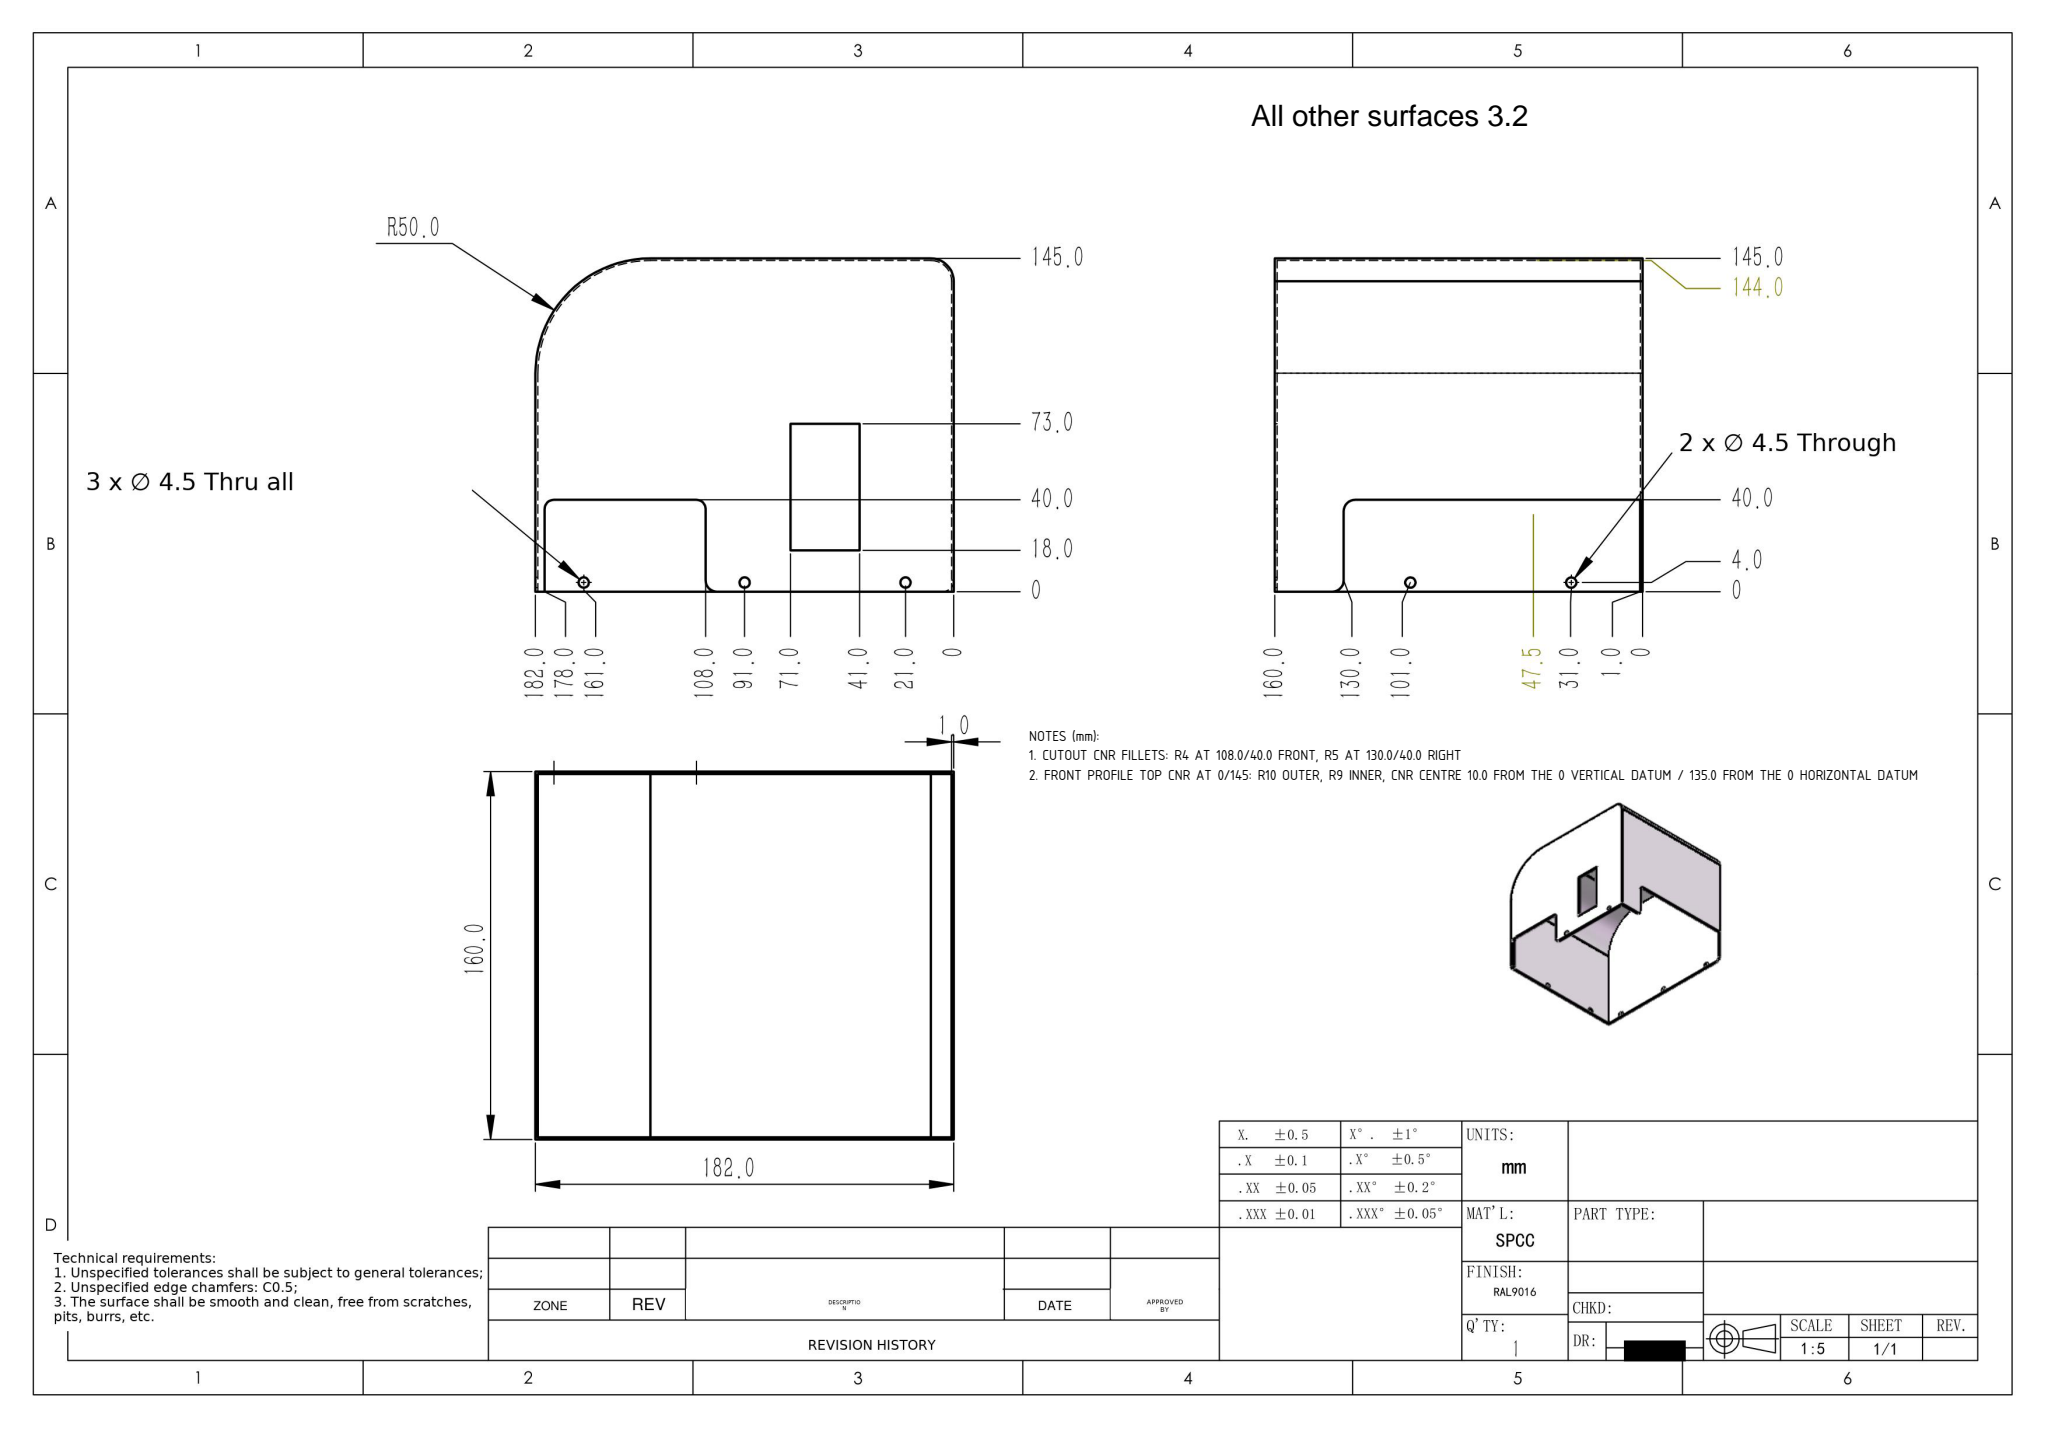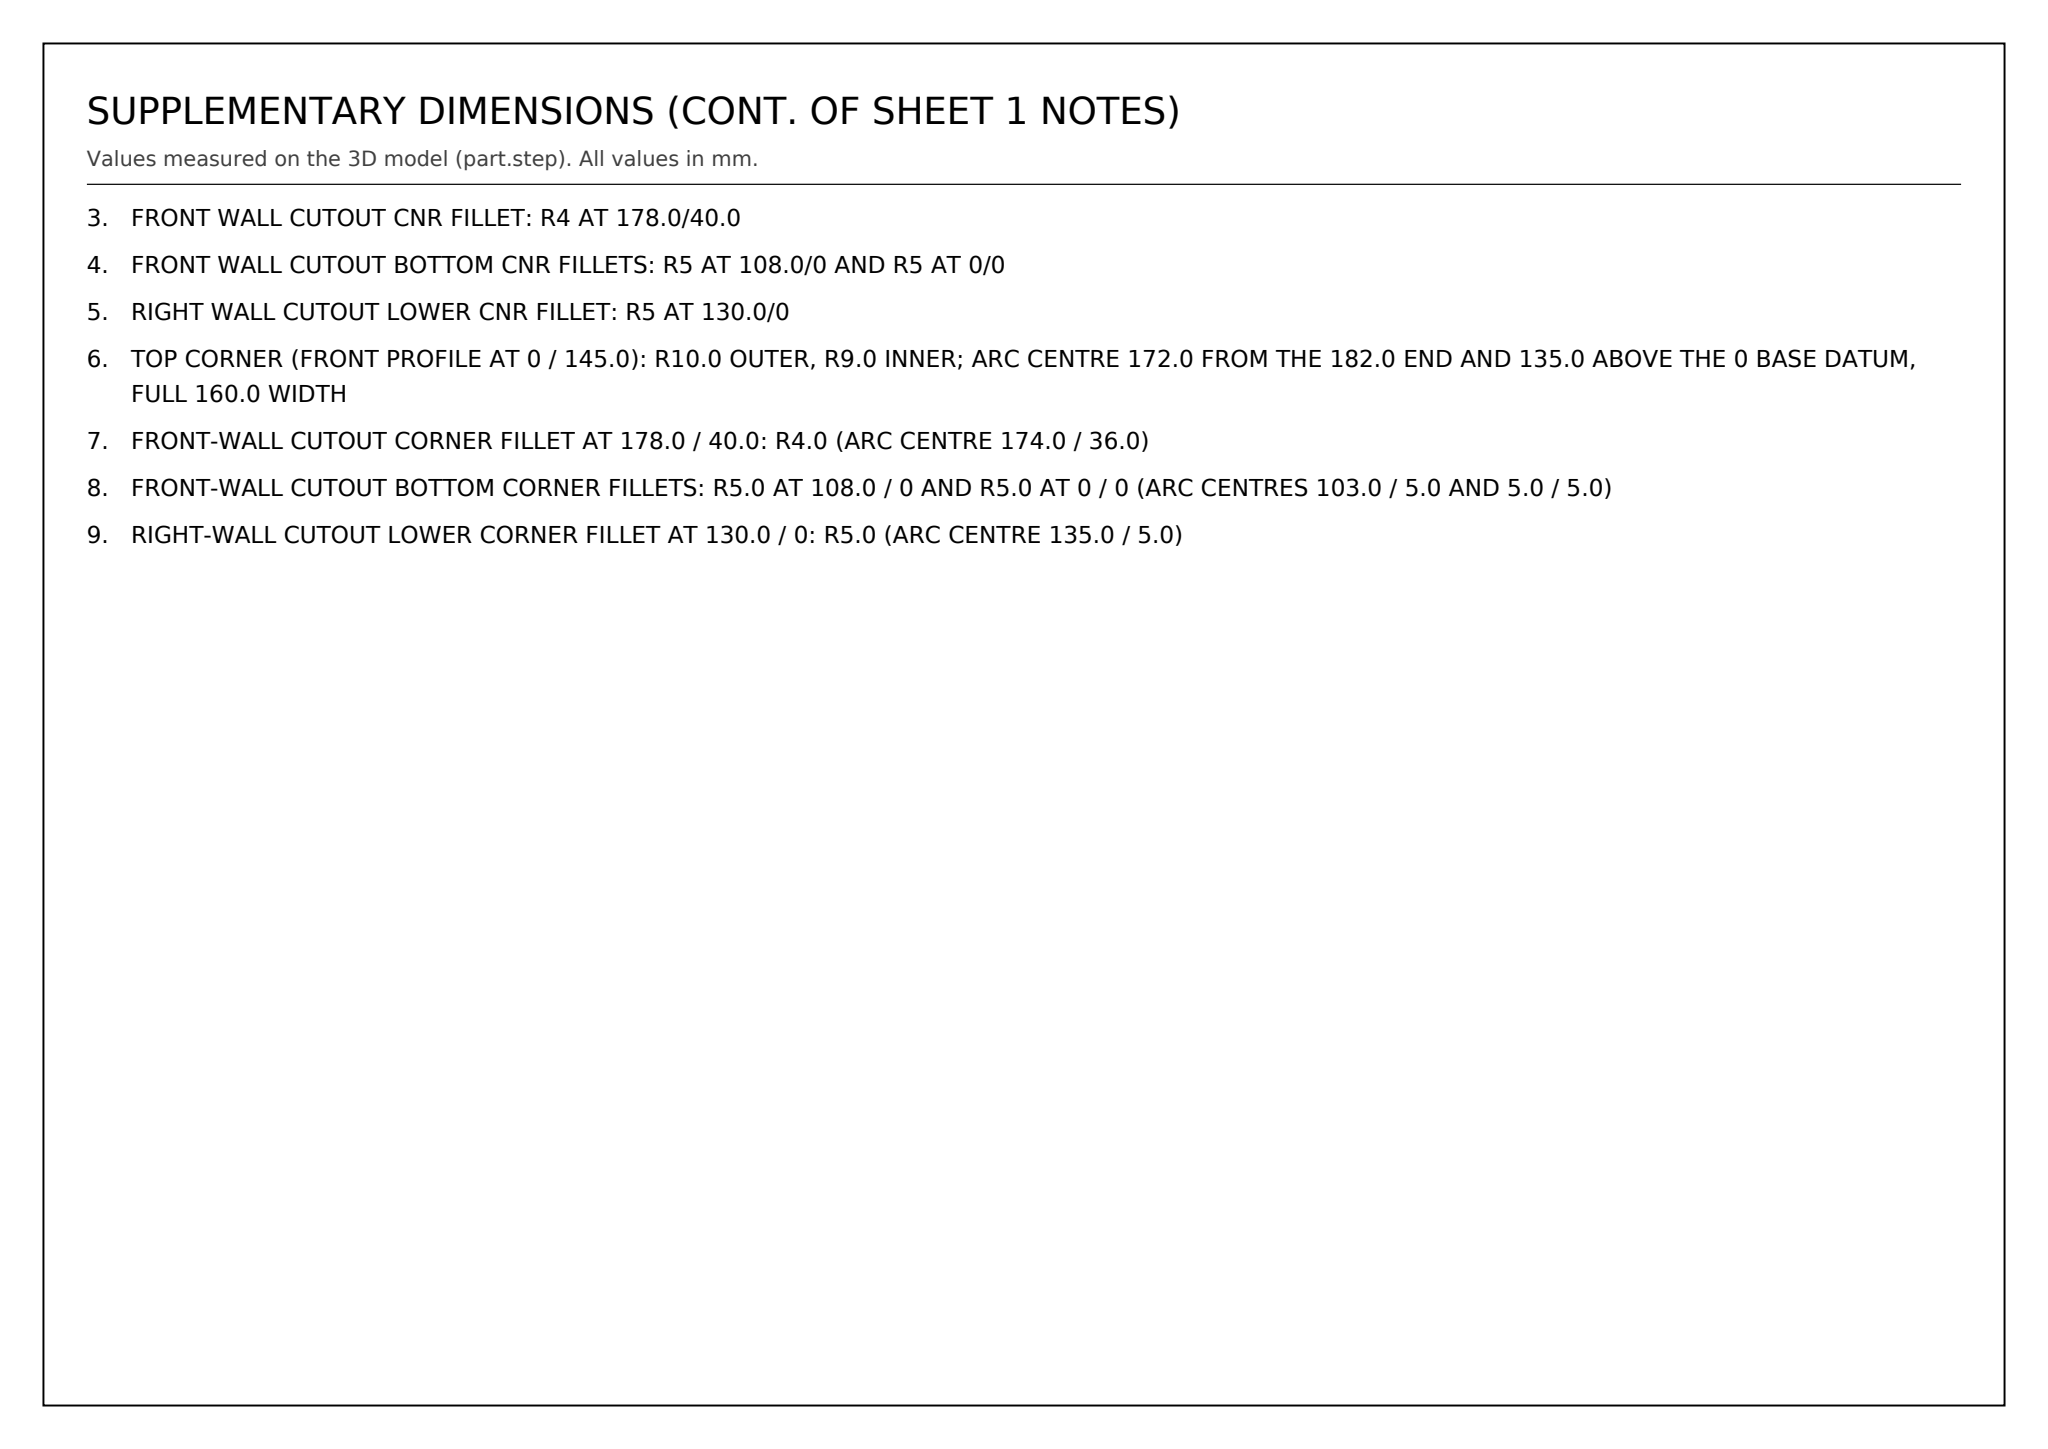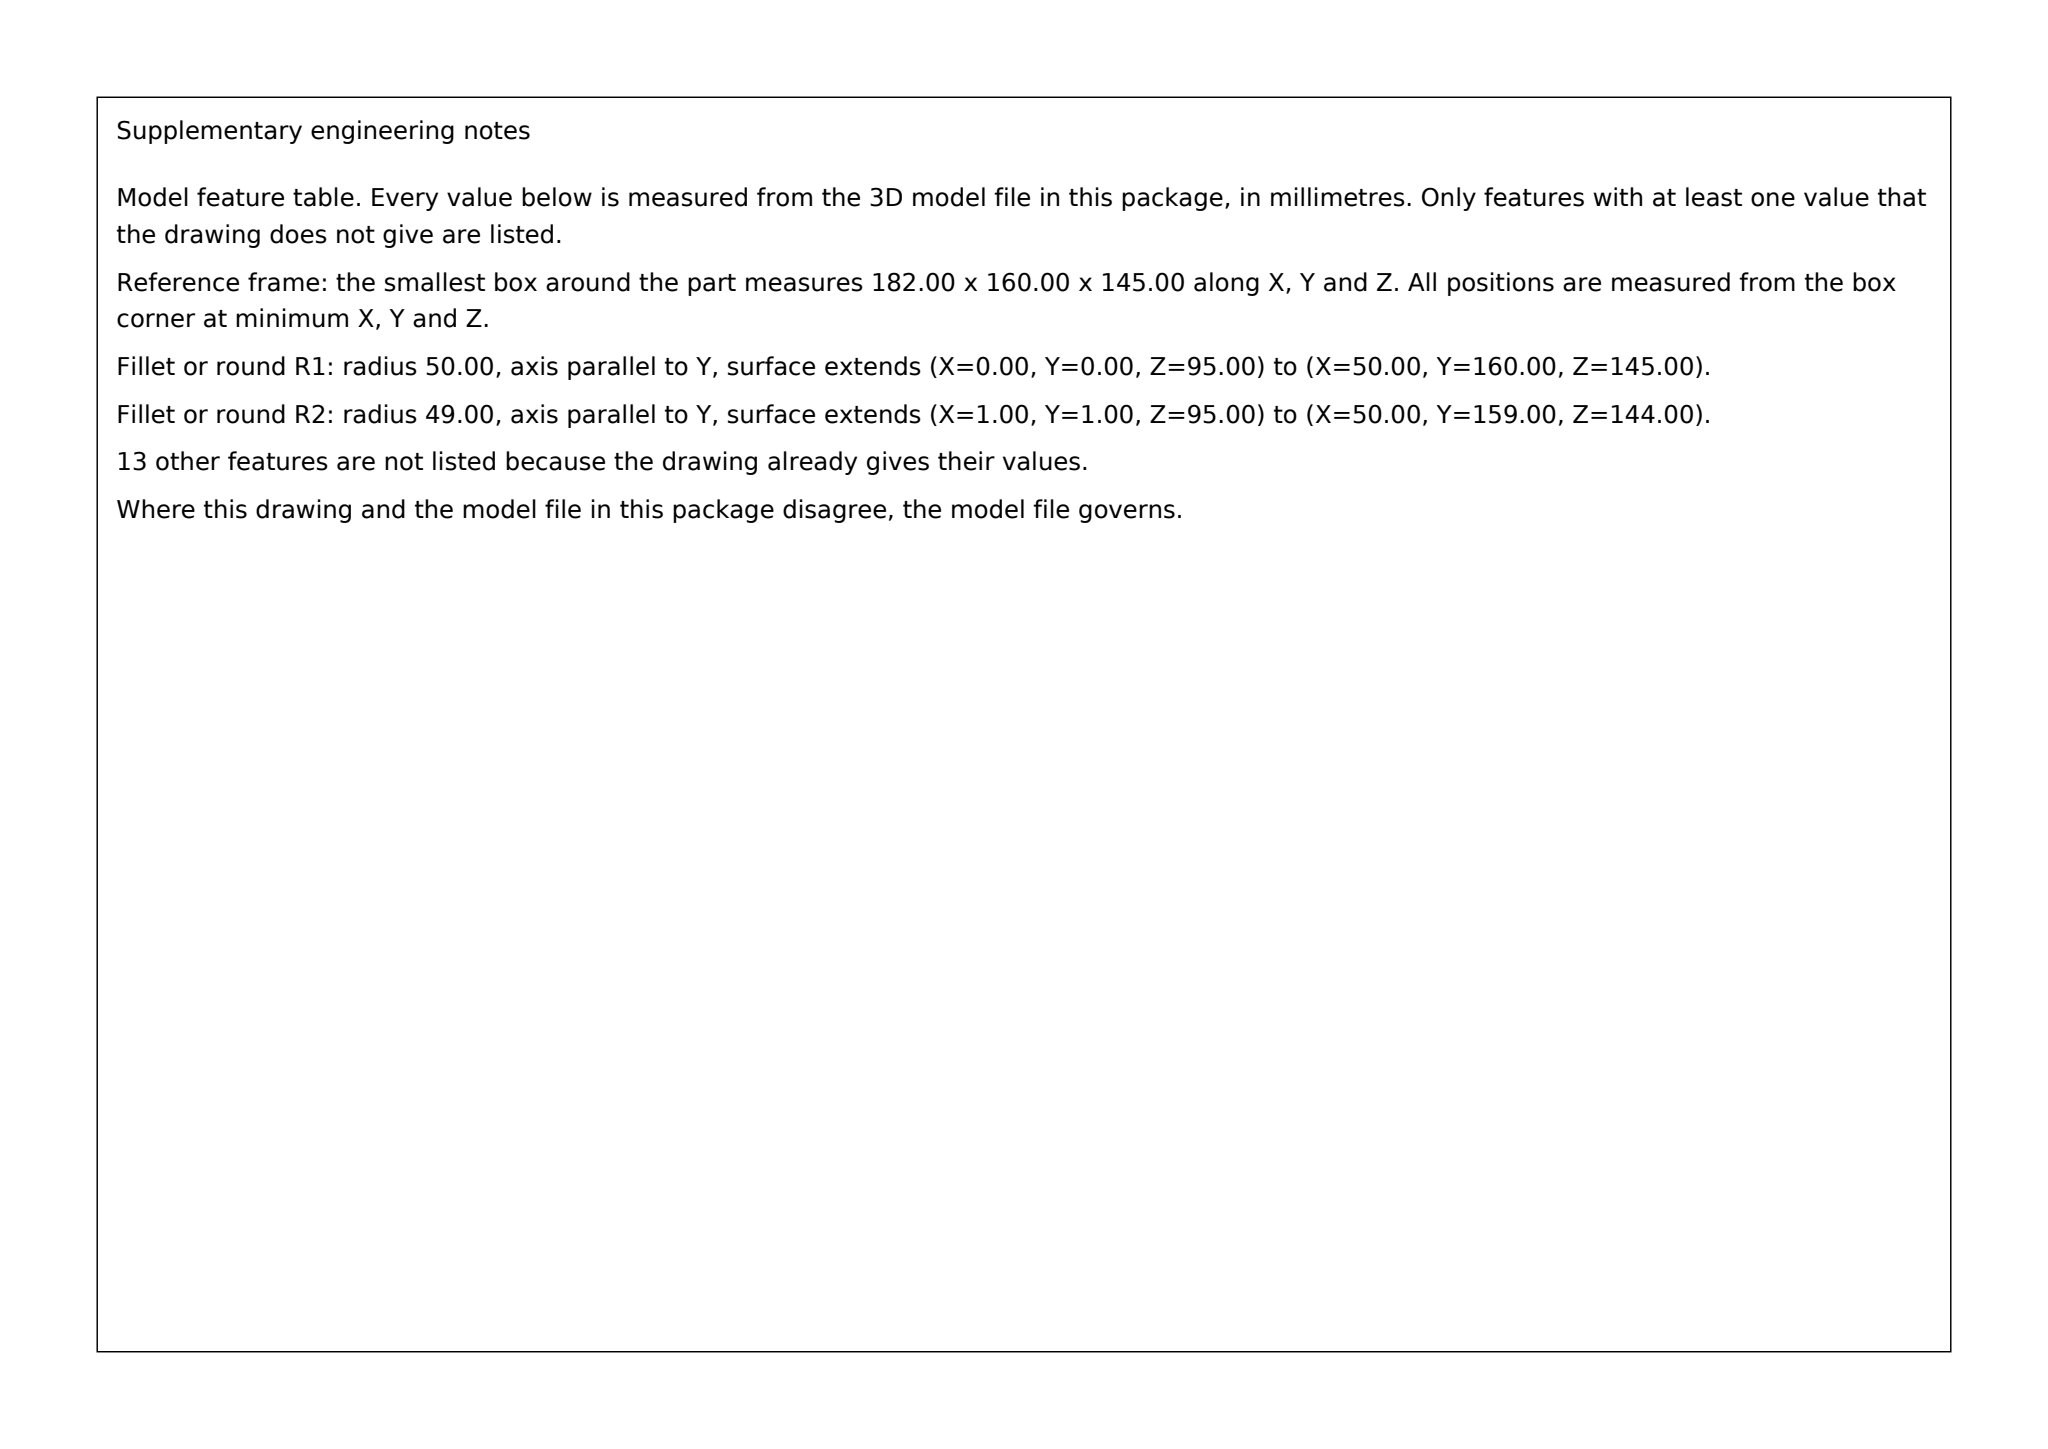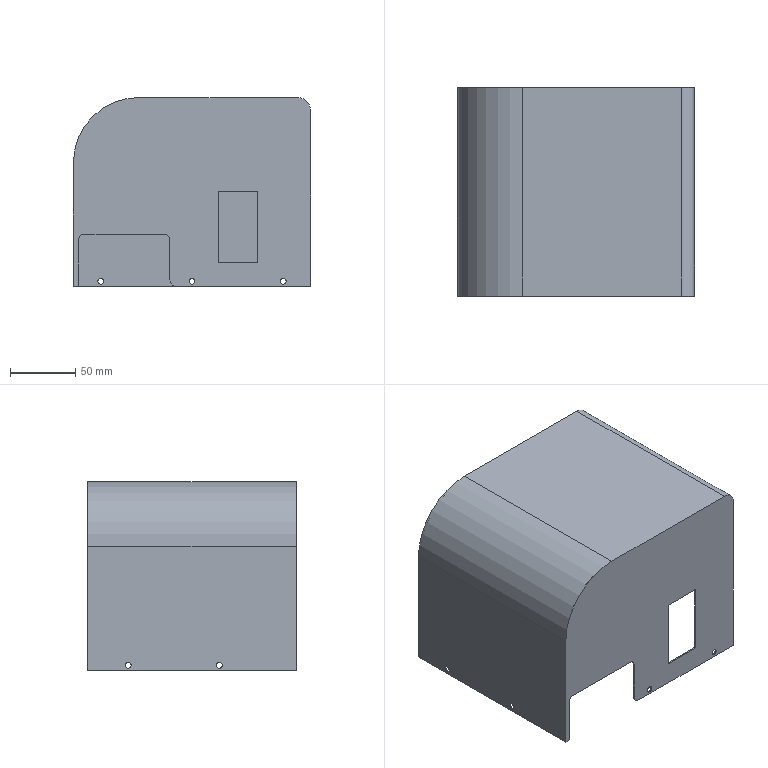Part | SolidWorks | mm | 1 solid | 45 faces | box 182 x 160 x 145 mm | volume 112198 mm3 | cylinder 24 | plane 21 | commonest cylinder face diameters 4.5 x14 10 x4 8 x2 100 x1 20 x1 98 x1 18 x1
Drawing notes:
CUTOUT CNR FILLETS: R4 AT 108.0/40.0 FRONT, R5 AT 130.0/40.0 RIGHT | from the solid: Y-axis cyl Ø8 at (x=70,z=36) tangent to planes x=74 & z=40 -> R4; drawing coord 182-74=108.0. X-axis cyl Ø10 at (y=35,z=35) tangent to planes y=30 & z=40 -> R5; drawing coord 160-30=130.0
FRONT PROFILE TOP CNR AT 0/145: R10 OUTER, R9 INNER, CNR CENTRE 10.0 FROM THE 0 VERTICAL DATUM / 135.0 FROM THE 0 HORIZONTAL DATUM | from the solid: cylinders dia 20.0 (L=160.0) and dia 18.0 (L=158.0), axis y, pos (172.0, 135.0)
FRONT WALL CUTOUT CNR FILLET: R4 AT 178.0/40.0 | from the solid: cylinder dia 8.0, axis y, pos (8.0, 36.0) = 182-8=174 -> tangent at 178.0/40.0
FRONT WALL CUTOUT BOTTOM CNR FILLETS: R5 AT 108.0/0 AND R5 AT 0/0 | from the solid: cylinders dia 10.0, axis y, pos (79.0, 5.0) and (177.0, 5.0)
RIGHT WALL CUTOUT LOWER CNR FILLET: R5 AT 130.0/0 | from the solid: cylinder dia 10.0, axis x, pos (y=25.0, z=5.0) -> tangent at 130.0/0
TOP CORNER (FRONT PROFILE AT 0 / 145.0): R10.0 OUTER, R9.0 INNER; ARC CENTRE 172.0 FROM THE 182.0 END AND 135.0 ABOVE THE 0 BASE DATUM, FULL 160.0 WIDTH | from the solid: cylinders dia 20.0 (len 160.0) and dia 18.0 (len 158.0), axis y, position [172.0, 135.0]
FRONT-WALL CUTOUT CORNER FILLET AT 178.0 / 40.0: R4.0 (ARC CENTRE 174.0 / 36.0) | from the solid: cylinder dia 8.0, axis y, position [8.0, 36.0] = 178.0/40.0 corner in front-view datum (x_draw = 182 - x_step)
FRONT-WALL CUTOUT BOTTOM CORNER FILLETS: R5.0 AT 108.0 / 0 AND R5.0 AT 0 / 0 (ARC CENTRES 103.0 / 5.0 AND 5.0 / 5.0) | from the solid: cylinders dia 10.0, axis y, positions [79.0, 5.0] and [177.0, 5.0]
RIGHT-WALL CUTOUT LOWER CORNER FILLET AT 130.0 / 0: R5.0 (ARC CENTRE 135.0 / 5.0) | from the solid: cylinder dia 10.0, axis x, position [y 25.0, z 5.0] = 130.0/0 corner in right-view datum (y_draw = 160 - y_step)
build123d program:
from build123d import *

# Parameters (mm, degrees)
SKETCH1_W            = 182
SKETCH1_H            = 160
BOSS_EXTRUDE1_DEPTH  = 145
FILLET1_R            = 50
FILLET3_R            = 10
SHELL1_T             = -1
SKETCH2_W            = 30
SKETCH2_H            = 55
CUT_EXTRUDE1_DEPTH   = 10
M4_CLEARANCE_HOLE2_D = 4.5
CUT_EXTRUDE2_REACH   = 248.067
SKETCH5_W            = 40
SKETCH5_H            = 129
M4_CLEARANCE_HOLE1_D = 4.5
FILLET2_R            = 5


with BuildPart() as part:
    # Sketch1 → Boss-Extrude1 (new body)
    with BuildSketch(Plane.XY):
        Rectangle(SKETCH1_W, SKETCH1_H)
    extrude(amount=BOSS_EXTRUDE1_DEPTH)

    # Fillet1
    fillet1_edges = [part.edges().sort_by_distance(p)[0] for p in [
        (-91, 0, 145),
    ]]
    fillet(fillet1_edges, radius=FILLET1_R)

    # Fillet3
    fillet3_edges = [part.edges().sort_by_distance(p)[0] for p in [
        (91, 0, 145),
    ]]
    fillet(fillet3_edges, radius=FILLET3_R)

    # Shell1
    shell1_openings = [part.faces().sort_by_distance(p)[0] for p in [
        (0, 0, 0),
    ]]
    offset(amount=SHELL1_T, openings=shell1_openings, kind=Kind.INTERSECTION)

    # Sketch2 → Cut-Extrude1 (cut)
    with BuildSketch(Plane.XZ.offset(80)):
        with BuildLine():
            Line((-87, 0), (-17, 0))
            Line((-17, 0), (-17, 36))
            ThreePointArc((-17, 36), (-18.172, 38.828), (-21, 40))
            Line((-21, 40), (-83, 40))
            ThreePointArc((-83, 40), (-85.828, 38.828), (-87, 36))
            Line((-87, 36), (-87, 0))
        make_face()
        with Locations((35, 45.5)):
            Rectangle(SKETCH2_W, SKETCH2_H)
    extrude(amount=-CUT_EXTRUDE1_DEPTH, mode=Mode.SUBTRACT)

    # M4 Clearance Hole2 (through all)
    with Locations(Plane.XZ.offset(80)):
        with Locations((-70, 4), (0, 4), (70, 4)):
            Hole(M4_CLEARANCE_HOLE2_D / 2)

    # Sketch5 → Cut-Extrude2 (cut, up to next)
    with BuildSketch(Plane(origin=(91, 0, 0), x_dir=(0, 0, -1), z_dir=(1, 0, 0)), mode=Mode.PRIVATE) as cut_extrude2_sk1:
        with Locations((-20, 14.5)):
            Rectangle(SKETCH5_W, SKETCH5_H)
    cut_extrude2_tool1 = extrude(cut_extrude2_sk1.sketch, amount=-CUT_EXTRUDE2_REACH, mode=Mode.PRIVATE) & part.part
    add(cut_extrude2_tool1.solids().sort_by_distance((91, 14.5, 20))[0], mode=Mode.SUBTRACT)

    # M4 Clearance Hole1 (through all)
    with Locations(Plane.ZY.offset(91)):
        with Locations((4, 49), (4, -21)):
            Hole(M4_CLEARANCE_HOLE1_D / 2)

    # Fillet2
    fillet2_edges = [part.edges().sort_by_distance(p)[0] for p in [
        (90.5, -50, 0),
        (-17, -79.5, 0),
        (91, 79.5, 0),
        (90.5, -50, 40),
    ]]
    fillet(fillet2_edges, radius=FILLET2_R)


solid = part.part